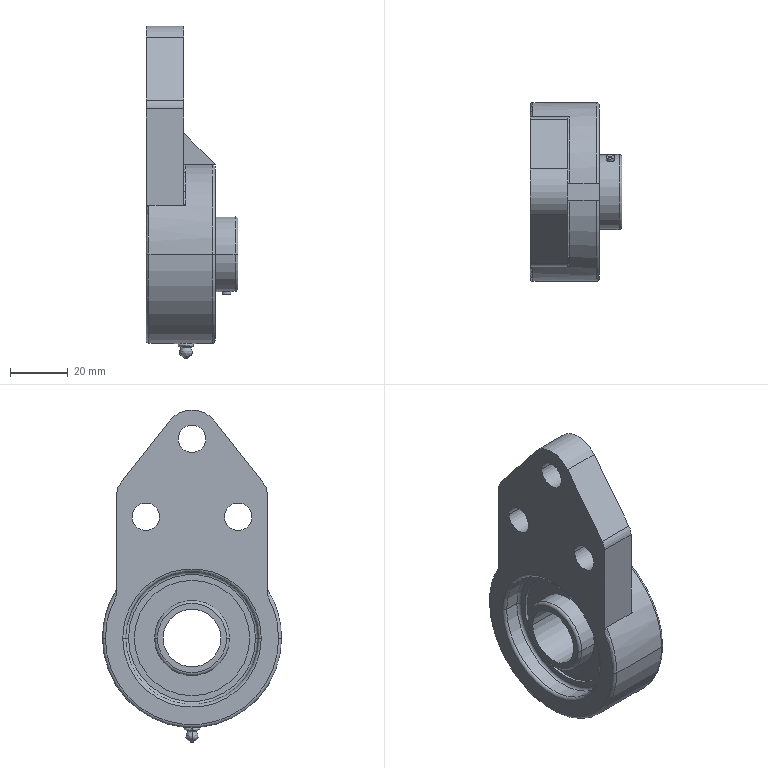Component | SolidWorks | CCDUCFB204-1 | 2 solids | 81 faces | volume 80109 mm3 | cylinder 39 | plane 20 | torus 18 | spline 4 | commonest cylinder face diameters 1 x7 26 x6 9.5 x6 3 x4 40 x4 46 x4 20 x3 62 x3 | material AISI 1045 Steel, Cold Drawn